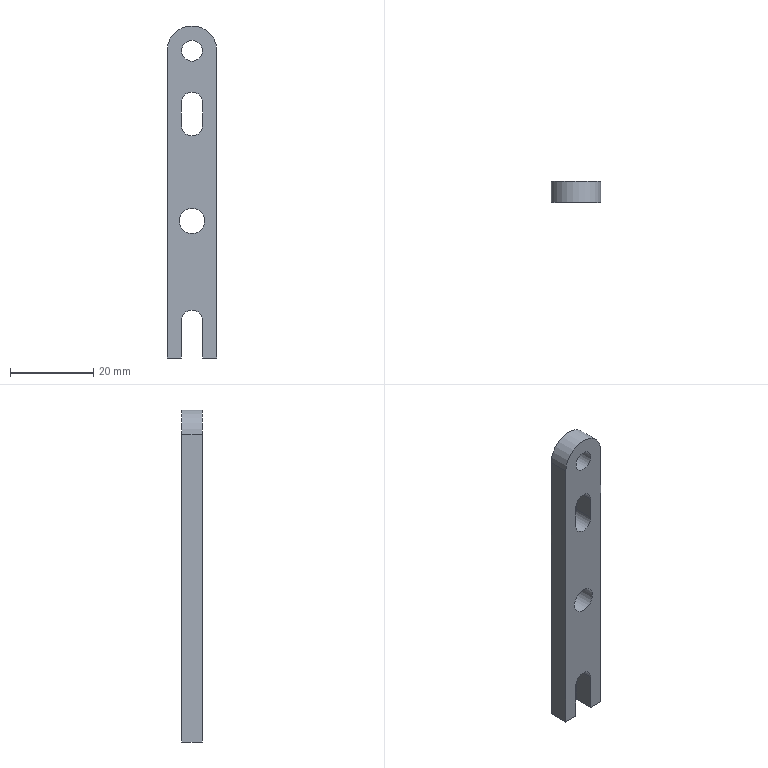Component | NX | BI_LINK | 1 solid | 16 faces | volume 3955 mm3 | plane 10 | cylinder 6 | commonest cylinder face diameters 5.1 x3 12 x1 5 x1 6.1 x1